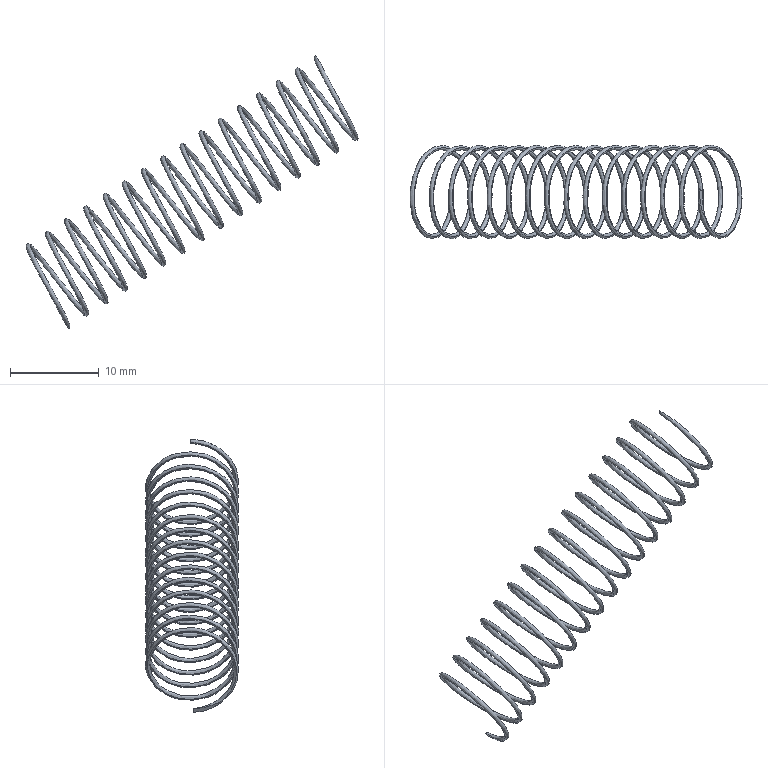Component | SolidWorks | HB362-65EndNotTightenedGroundFlat0.25Turns10x50-1 | 1 solid | 6 faces | volume 96 mm3 | plane 4 | spline 2 | material Carbon Spring Steel Wire